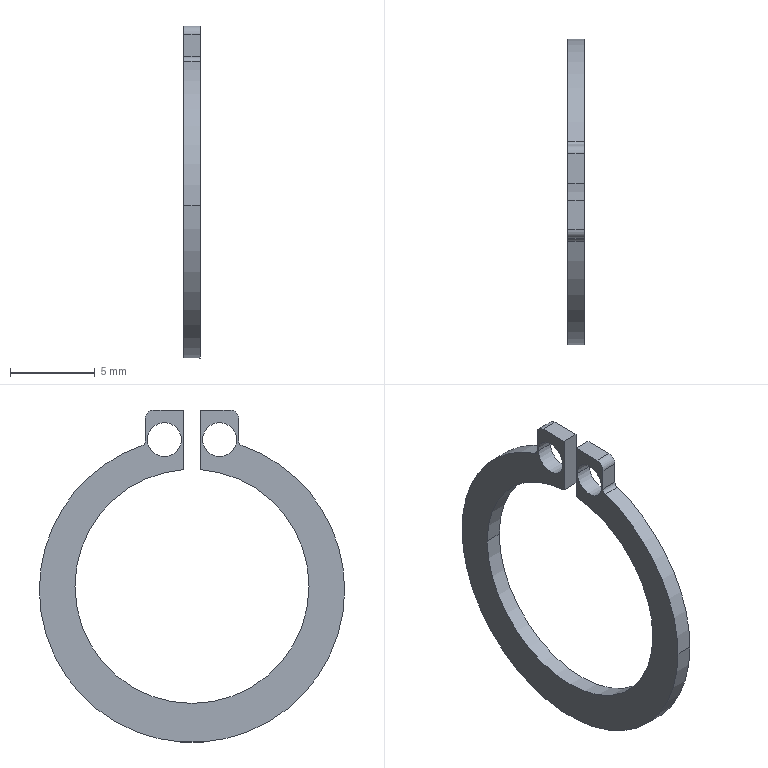Component | SolidWorks | CCD11-00TensioningAssembly-2_CCDAxisCard15-1 | 1 solid | 22 faces | box 1 x 18 x 19.6 mm | volume 105 mm3 | cylinder 14 | plane 8 | commonest cylinder face diameters 2 x4 18 x3 13.8 x3 1 x2 0.6 x2
build123d program:
from build123d import *

# Parameters (mm, degrees)
SKETCH1_R           = 1
BOSS_EXTRUDE1_DEPTH = 1


with BuildPart() as part:
    # Sketch1 → Boss-Extrude1 (new body)
    with BuildSketch(Plane.XY.offset(1)):
        with BuildLine():
            Line((2.75, -9.9), (2.75, -8.586))
            ThreePointArc((2.75, -8.586), (2.806, -8.412), (2.952, -8.302))
            ThreePointArc((2.952, -8.302), (0, 9.2), (-2.952, -8.302))
            ThreePointArc((-2.952, -8.302), (-2.806, -8.412), (-2.75, -8.586))
            Line((-2.75, -8.586), (-2.75, -9.9))
            ThreePointArc((-2.75, -9.9), (-2.604, -10.254), (-2.25, -10.4))
            Line((-2.25, -10.4), (-0.5, -10.4))
            Line((-0.5, -10.4), (-0.5, -6.882))
            ThreePointArc((-0.5, -6.882), (0, 6.9), (0.5, -6.882))
            Line((0.5, -6.882), (0.5, -10.4))
            Line((0.5, -10.4), (2.25, -10.4))
            ThreePointArc((2.25, -10.4), (2.604, -10.254), (2.75, -9.9))
        make_face()
        with Locations(Location((1.625, -8.65, 0), (0, 0, 180))):
            Circle(SKETCH1_R, mode=Mode.SUBTRACT)
        with Locations(Location((-1.625, -8.65, 0), (0, 0, 180))):
            Circle(SKETCH1_R, mode=Mode.SUBTRACT)
    extrude(amount=-BOSS_EXTRUDE1_DEPTH)


solid = part.part

# Placed as in the assembly
solid = solid.moved(Location((119.879, 107.251, 149), (-90, 90, 0)))
STEP:
#1=COLOUR_RGB('',0.7922,0.8196,0.9333);
#2=FILL_AREA_STYLE_COLOUR('',#1);
#3=FILL_AREA_STYLE('',(#2));
#4=SURFACE_STYLE_FILL_AREA(#3);
#5=SURFACE_SIDE_STYLE('',(#4));
#6=SURFACE_STYLE_USAGE(.BOTH.,#5);
#7=PRESENTATION_STYLE_ASSIGNMENT((#6));
#8=CARTESIAN_POINT('',(4.759,4.119,6.207));
#9=VERTEX_POINT('',#8);
#10=CARTESIAN_POINT('',(4.759,4.198,6.207));
#11=VERTEX_POINT('',#10);
#12=CARTESIAN_POINT('',(4.759,4.159,6.207));
#13=DIRECTION('',(-1.,-0.,0.));
#14=DIRECTION('',(0.,-1.,0.));
#15=AXIS2_PLACEMENT_3D('',#12,#13,#14);
#16=CIRCLE('',#15,0.03937);
#17=EDGE_CURVE('',#9,#11,#16,.T.);
#18=ORIENTED_EDGE('',*,*,#17,.F.);
#19=CARTESIAN_POINT('',(4.72,4.119,6.207));
#20=VERTEX_POINT('',#19);
#21=CARTESIAN_POINT('',(4.759,4.119,6.207));
#22=DIRECTION('',(-1.,-0.,0.));
#23=VECTOR('',#22,39.37);
#24=LINE('',#21,#23);
#25=EDGE_CURVE('',#9,#20,#24,.T.);
#26=ORIENTED_EDGE('',*,*,#25,.T.);
#27=CARTESIAN_POINT('',(4.72,4.198,6.207));
#28=VERTEX_POINT('',#27);
#29=CARTESIAN_POINT('',(4.72,4.159,6.207));
#30=DIRECTION('',(-1.,-0.,0.));
#31=DIRECTION('',(0.,-1.,0.));
#32=AXIS2_PLACEMENT_3D('',#29,#30,#31);
#33=CIRCLE('',#32,0.03937);
#34=EDGE_CURVE('',#20,#28,#33,.T.);
#35=ORIENTED_EDGE('',*,*,#34,.T.);
#36=CARTESIAN_POINT('',(4.759,4.198,6.207));
#37=DIRECTION('',(-1.,-0.,0.));
#38=VECTOR('',#37,39.37);
#39=LINE('',#36,#38);
#40=EDGE_CURVE('',#11,#28,#39,.T.);
#41=ORIENTED_EDGE('',*,*,#40,.F.);
#42=EDGE_LOOP('',(#18,#26,#35,#41));
#43=FACE_OUTER_BOUND('',#42,.T.);
#44=CARTESIAN_POINT('',(4.759,4.159,6.207));
#45=DIRECTION('',(-1.,-0.,0.));
#46=DIRECTION('',(0.,1.,0.));
#47=AXIS2_PLACEMENT_3D('',#44,#45,#46);
#48=CYLINDRICAL_SURFACE('',#47,0.03937);
#49=ADVANCED_FACE('',(#43),#48,.F.);
#50=CARTESIAN_POINT('',(4.759,4.247,6.207));
#51=VERTEX_POINT('',#50);
#52=CARTESIAN_POINT('',(4.759,4.326,6.207));
#53=VERTEX_POINT('',#52);
#54=CARTESIAN_POINT('',(4.759,4.286,6.207));
#55=DIRECTION('',(-1.,-0.,0.));
#56=DIRECTION('',(0.,-1.,0.));
#57=AXIS2_PLACEMENT_3D('',#54,#55,#56);
#58=CIRCLE('',#57,0.03937);
#59=EDGE_CURVE('',#51,#53,#58,.T.);
#60=ORIENTED_EDGE('',*,*,#59,.F.);
#61=CARTESIAN_POINT('',(4.72,4.247,6.207));
#62=VERTEX_POINT('',#61);
#63=CARTESIAN_POINT('',(4.759,4.247,6.207));
#64=DIRECTION('',(-1.,-0.,0.));
#65=VECTOR('',#64,39.37);
#66=LINE('',#63,#65);
#67=EDGE_CURVE('',#51,#62,#66,.T.);
#68=ORIENTED_EDGE('',*,*,#67,.T.);
#69=CARTESIAN_POINT('',(4.72,4.326,6.207));
#70=VERTEX_POINT('',#69);
#71=CARTESIAN_POINT('',(4.72,4.286,6.207));
#72=DIRECTION('',(-1.,-0.,0.));
#73=DIRECTION('',(0.,-1.,0.));
#74=AXIS2_PLACEMENT_3D('',#71,#72,#73);
#75=CIRCLE('',#74,0.03937);
#76=EDGE_CURVE('',#62,#70,#75,.T.);
#77=ORIENTED_EDGE('',*,*,#76,.T.);
#78=CARTESIAN_POINT('',(4.759,4.326,6.207));
#79=DIRECTION('',(-1.,-0.,0.));
#80=VECTOR('',#79,39.37);
#81=LINE('',#78,#80);
#82=EDGE_CURVE('',#53,#70,#81,.T.);
#83=ORIENTED_EDGE('',*,*,#82,.F.);
#84=EDGE_LOOP('',(#60,#68,#77,#83));
#85=FACE_OUTER_BOUND('',#84,.T.);
#86=CARTESIAN_POINT('',(4.759,4.286,6.207));
#87=DIRECTION('',(-1.,-0.,0.));
#88=DIRECTION('',(0.,1.,0.));
#89=AXIS2_PLACEMENT_3D('',#86,#87,#88);
#90=CYLINDRICAL_SURFACE('',#89,0.03937);
#91=ADVANCED_FACE('',(#85),#90,.F.);
#92=CARTESIAN_POINT('',(4.759,4.577,5.858));
#93=VERTEX_POINT('',#92);
#94=CARTESIAN_POINT('',(4.759,3.868,5.858));
#95=VERTEX_POINT('',#94);
#96=CARTESIAN_POINT('',(4.759,4.222,5.858));
#97=DIRECTION('',(-1.,-0.,0.));
#98=DIRECTION('',(-0.,1.,0.));
#99=AXIS2_PLACEMENT_3D('',#96,#97,#98);
#100=CIRCLE('',#99,0.3543);
#101=EDGE_CURVE('',#93,#95,#100,.T.);
#102=ORIENTED_EDGE('',*,*,#101,.T.);
#103=CARTESIAN_POINT('',(4.72,3.868,5.858));
#104=VERTEX_POINT('',#103);
#105=CARTESIAN_POINT('',(4.759,3.868,5.858));
#106=DIRECTION('',(-1.,-0.,0.));
#107=VECTOR('',#106,39.37);
#108=LINE('',#105,#107);
#109=EDGE_CURVE('',#95,#104,#108,.T.);
#110=ORIENTED_EDGE('',*,*,#109,.T.);
#111=CARTESIAN_POINT('',(4.72,4.577,5.858));
#112=VERTEX_POINT('',#111);
#113=CARTESIAN_POINT('',(4.72,4.222,5.858));
#114=DIRECTION('',(-1.,-0.,0.));
#115=DIRECTION('',(-0.,1.,0.));
#116=AXIS2_PLACEMENT_3D('',#113,#114,#115);
#117=CIRCLE('',#116,0.3543);
#118=EDGE_CURVE('',#112,#104,#117,.T.);
#119=ORIENTED_EDGE('',*,*,#118,.F.);
#120=CARTESIAN_POINT('',(4.759,4.577,5.858));
#121=DIRECTION('',(-1.,-0.,0.));
#122=VECTOR('',#121,39.37);
#123=LINE('',#120,#122);
#124=EDGE_CURVE('',#93,#112,#123,.T.);
#125=ORIENTED_EDGE('',*,*,#124,.F.);
#126=EDGE_LOOP('',(#102,#110,#119,#125));
#127=FACE_OUTER_BOUND('',#126,.T.);
#128=CARTESIAN_POINT('',(4.759,4.222,5.858));
#129=DIRECTION('',(-1.,-0.,0.));
#130=DIRECTION('',(-0.,1.,0.));
#131=AXIS2_PLACEMENT_3D('',#128,#129,#130);
#132=CYLINDRICAL_SURFACE('',#131,0.3543);
#133=ADVANCED_FACE('',(#127),#132,.T.);
#134=CARTESIAN_POINT('',(4.759,4.339,6.193));
#135=VERTEX_POINT('',#134);
#136=CARTESIAN_POINT('',(4.759,4.222,5.858));
#137=DIRECTION('',(-1.,-0.,0.));
#138=DIRECTION('',(-0.,1.,0.));
#139=AXIS2_PLACEMENT_3D('',#136,#137,#138);
#140=CIRCLE('',#139,0.3543);
#141=EDGE_CURVE('',#135,#93,#140,.T.);
#142=ORIENTED_EDGE('',*,*,#141,.T.);
#143=ORIENTED_EDGE('',*,*,#124,.T.);
#144=CARTESIAN_POINT('',(4.72,4.339,6.193));
#145=VERTEX_POINT('',#144);
#146=CARTESIAN_POINT('',(4.72,4.222,5.858));
#147=DIRECTION('',(-1.,-0.,0.));
#148=DIRECTION('',(-0.,1.,0.));
#149=AXIS2_PLACEMENT_3D('',#146,#147,#148);
#150=CIRCLE('',#149,0.3543);
#151=EDGE_CURVE('',#145,#112,#150,.T.);
#152=ORIENTED_EDGE('',*,*,#151,.F.);
#153=CARTESIAN_POINT('',(4.759,4.339,6.193));
#154=DIRECTION('',(-1.,-0.,0.));
#155=VECTOR('',#154,39.37);
#156=LINE('',#153,#155);
#157=EDGE_CURVE('',#135,#145,#156,.T.);
#158=ORIENTED_EDGE('',*,*,#157,.F.);
#159=EDGE_LOOP('',(#142,#143,#152,#158));
#160=FACE_OUTER_BOUND('',#159,.T.);
#161=CARTESIAN_POINT('',(4.759,4.222,5.858));
#162=DIRECTION('',(-1.,-0.,0.));
#163=DIRECTION('',(-0.,1.,0.));
#164=AXIS2_PLACEMENT_3D('',#161,#162,#163);
#165=CYLINDRICAL_SURFACE('',#164,0.3543);
#166=ADVANCED_FACE('',(#160),#165,.T.);
#167=CARTESIAN_POINT('',(4.759,4.203,6.137));
#168=VERTEX_POINT('',#167);
#169=CARTESIAN_POINT('',(4.759,3.951,5.866));
#170=VERTEX_POINT('',#169);
#171=CARTESIAN_POINT('',(4.759,4.222,5.866));
#172=DIRECTION('',(1.,0.,-0.));
#173=DIRECTION('',(0.,-1.,0.));
#174=AXIS2_PLACEMENT_3D('',#171,#172,#173);
#175=CIRCLE('',#174,0.2717);
#176=EDGE_CURVE('',#168,#170,#175,.T.);
#177=ORIENTED_EDGE('',*,*,#176,.T.);
#178=CARTESIAN_POINT('',(4.72,3.951,5.866));
#179=VERTEX_POINT('',#178);
#180=CARTESIAN_POINT('',(4.759,3.951,5.866));
#181=DIRECTION('',(-1.,-0.,0.));
#182=VECTOR('',#181,39.37);
#183=LINE('',#180,#182);
#184=EDGE_CURVE('',#170,#179,#183,.T.);
#185=ORIENTED_EDGE('',*,*,#184,.T.);
#186=CARTESIAN_POINT('',(4.72,4.203,6.137));
#187=VERTEX_POINT('',#186);
#188=CARTESIAN_POINT('',(4.72,4.222,5.866));
#189=DIRECTION('',(1.,0.,-0.));
#190=DIRECTION('',(0.,-1.,0.));
#191=AXIS2_PLACEMENT_3D('',#188,#189,#190);
#192=CIRCLE('',#191,0.2717);
#193=EDGE_CURVE('',#187,#179,#192,.T.);
#194=ORIENTED_EDGE('',*,*,#193,.F.);
#195=CARTESIAN_POINT('',(4.759,4.203,6.137));
#196=DIRECTION('',(-1.,-0.,0.));
#197=VECTOR('',#196,39.37);
#198=LINE('',#195,#197);
#199=EDGE_CURVE('',#168,#187,#198,.T.);
#200=ORIENTED_EDGE('',*,*,#199,.F.);
#201=EDGE_LOOP('',(#177,#185,#194,#200));
#202=FACE_OUTER_BOUND('',#201,.T.);
#203=CARTESIAN_POINT('',(4.759,4.222,5.866));
#204=DIRECTION('',(-1.,-0.,0.));
#205=DIRECTION('',(-0.,1.,0.));
#206=AXIS2_PLACEMENT_3D('',#203,#204,#205);
#207=CYLINDRICAL_SURFACE('',#206,0.2717);
#208=ADVANCED_FACE('',(#202),#207,.F.);
#209=ORIENTED_EDGE('',*,*,#184,.F.);
#210=CARTESIAN_POINT('',(4.759,4.494,5.866));
#211=VERTEX_POINT('',#210);
#212=CARTESIAN_POINT('',(4.759,4.222,5.866));
#213=DIRECTION('',(1.,0.,-0.));
#214=DIRECTION('',(0.,-1.,0.));
#215=AXIS2_PLACEMENT_3D('',#212,#213,#214);
#216=CIRCLE('',#215,0.2717);
#217=EDGE_CURVE('',#170,#211,#216,.T.);
#218=ORIENTED_EDGE('',*,*,#217,.T.);
#219=CARTESIAN_POINT('',(4.72,4.494,5.866));
#220=VERTEX_POINT('',#219);
#221=CARTESIAN_POINT('',(4.759,4.494,5.866));
#222=DIRECTION('',(-1.,-0.,0.));
#223=VECTOR('',#222,39.37);
#224=LINE('',#221,#223);
#225=EDGE_CURVE('',#211,#220,#224,.T.);
#226=ORIENTED_EDGE('',*,*,#225,.T.);
#227=CARTESIAN_POINT('',(4.72,4.222,5.866));
#228=DIRECTION('',(1.,0.,-0.));
#229=DIRECTION('',(0.,-1.,0.));
#230=AXIS2_PLACEMENT_3D('',#227,#228,#229);
#231=CIRCLE('',#230,0.2717);
#232=EDGE_CURVE('',#179,#220,#231,.T.);
#233=ORIENTED_EDGE('',*,*,#232,.F.);
#234=EDGE_LOOP('',(#209,#218,#226,#233));
#235=FACE_OUTER_BOUND('',#234,.T.);
#236=CARTESIAN_POINT('',(4.759,4.222,5.866));
#237=DIRECTION('',(-1.,-0.,0.));
#238=DIRECTION('',(-0.,1.,0.));
#239=AXIS2_PLACEMENT_3D('',#236,#237,#238);
#240=CYLINDRICAL_SURFACE('',#239,0.2717);
#241=ADVANCED_FACE('',(#235),#240,.F.);
#242=CARTESIAN_POINT('',(4.72,4.311,6.276));
#243=VERTEX_POINT('',#242);
#244=CARTESIAN_POINT('',(4.72,4.331,6.256));
#245=VERTEX_POINT('',#244);
#246=CARTESIAN_POINT('',(4.72,4.311,6.256));
#247=DIRECTION('',(-1.,-0.,0.));
#248=DIRECTION('',(0.,1.,0.));
#249=AXIS2_PLACEMENT_3D('',#246,#247,#248);
#250=CIRCLE('',#249,0.01969);
#251=EDGE_CURVE('',#243,#245,#250,.T.);
#252=ORIENTED_EDGE('',*,*,#251,.F.);
#253=CARTESIAN_POINT('',(4.759,4.311,6.276));
#254=VERTEX_POINT('',#253);
#255=CARTESIAN_POINT('',(4.759,4.311,6.276));
#256=DIRECTION('',(-1.,-0.,0.));
#257=VECTOR('',#256,39.37);
#258=LINE('',#255,#257);
#259=EDGE_CURVE('',#254,#243,#258,.T.);
#260=ORIENTED_EDGE('',*,*,#259,.F.);
#261=CARTESIAN_POINT('',(4.759,4.331,6.256));
#262=VERTEX_POINT('',#261);
#263=CARTESIAN_POINT('',(4.759,4.311,6.256));
#264=DIRECTION('',(-1.,-0.,0.));
#265=DIRECTION('',(0.,1.,0.));
#266=AXIS2_PLACEMENT_3D('',#263,#264,#265);
#267=CIRCLE('',#266,0.01969);
#268=EDGE_CURVE('',#254,#262,#267,.T.);
#269=ORIENTED_EDGE('',*,*,#268,.T.);
#270=CARTESIAN_POINT('',(4.759,4.331,6.256));
#271=DIRECTION('',(-1.,-0.,0.));
#272=VECTOR('',#271,39.37);
#273=LINE('',#270,#272);
#274=EDGE_CURVE('',#262,#245,#273,.T.);
#275=ORIENTED_EDGE('',*,*,#274,.T.);
#276=EDGE_LOOP('',(#252,#260,#269,#275));
#277=FACE_OUTER_BOUND('',#276,.T.);
#278=CARTESIAN_POINT('',(4.759,4.311,6.256));
#279=DIRECTION('',(-1.,-0.,0.));
#280=DIRECTION('',(0.,1.,0.));
#281=AXIS2_PLACEMENT_3D('',#278,#279,#280);
#282=CYLINDRICAL_SURFACE('',#281,0.01969);
#283=ADVANCED_FACE('',(#277),#282,.T.);
#284=CARTESIAN_POINT('',(4.72,4.242,6.276));
#285=VERTEX_POINT('',#284);
#286=CARTESIAN_POINT('',(4.72,4.242,6.276));
#287=DIRECTION('',(-0.,1.,0.));
#288=VECTOR('',#287,39.37);
#289=LINE('',#286,#288);
#290=EDGE_CURVE('',#285,#243,#289,.T.);
#291=ORIENTED_EDGE('',*,*,#290,.F.);
#292=CARTESIAN_POINT('',(4.759,4.242,6.276));
#293=VERTEX_POINT('',#292);
#294=CARTESIAN_POINT('',(4.759,4.242,6.276));
#295=DIRECTION('',(-1.,-0.,0.));
#296=VECTOR('',#295,39.37);
#297=LINE('',#294,#296);
#298=EDGE_CURVE('',#293,#285,#297,.T.);
#299=ORIENTED_EDGE('',*,*,#298,.F.);
#300=CARTESIAN_POINT('',(4.759,4.242,6.276));
#301=DIRECTION('',(-0.,1.,0.));
#302=VECTOR('',#301,39.37);
#303=LINE('',#300,#302);
#304=EDGE_CURVE('',#293,#254,#303,.T.);
#305=ORIENTED_EDGE('',*,*,#304,.T.);
#306=ORIENTED_EDGE('',*,*,#259,.T.);
#307=EDGE_LOOP('',(#291,#299,#305,#306));
#308=FACE_OUTER_BOUND('',#307,.T.);
#309=CARTESIAN_POINT('',(4.759,4.242,6.276));
#310=DIRECTION('',(0.,-0.,1.));
#311=DIRECTION('',(-0.,1.,0.));
#312=AXIS2_PLACEMENT_3D('',#309,#310,#311);
#313=PLANE('',#312);
#314=ADVANCED_FACE('',(#308),#313,.T.);
#315=CARTESIAN_POINT('',(4.72,4.242,6.137));
#316=VERTEX_POINT('',#315);
#317=CARTESIAN_POINT('',(4.72,4.242,6.137));
#318=DIRECTION('',(0.,-0.,1.));
#319=VECTOR('',#318,39.37);
#320=LINE('',#317,#319);
#321=EDGE_CURVE('',#316,#285,#320,.T.);
#322=ORIENTED_EDGE('',*,*,#321,.F.);
#323=CARTESIAN_POINT('',(4.759,4.242,6.137));
#324=VERTEX_POINT('',#323);
#325=CARTESIAN_POINT('',(4.759,4.242,6.137));
#326=DIRECTION('',(-1.,-0.,0.));
#327=VECTOR('',#326,39.37);
#328=LINE('',#325,#327);
#329=EDGE_CURVE('',#324,#316,#328,.T.);
#330=ORIENTED_EDGE('',*,*,#329,.F.);
#331=CARTESIAN_POINT('',(4.759,4.242,6.137));
#332=DIRECTION('',(0.,-0.,1.));
#333=VECTOR('',#332,39.37);
#334=LINE('',#331,#333);
#335=EDGE_CURVE('',#324,#293,#334,.T.);
#336=ORIENTED_EDGE('',*,*,#335,.T.);
#337=ORIENTED_EDGE('',*,*,#298,.T.);
#338=EDGE_LOOP('',(#322,#330,#336,#337));
#339=FACE_OUTER_BOUND('',#338,.T.);
#340=CARTESIAN_POINT('',(4.759,4.242,6.137));
#341=DIRECTION('',(0.,-1.,-0.));
#342=DIRECTION('',(0.,-0.,1.));
#343=AXIS2_PLACEMENT_3D('',#340,#341,#342);
#344=PLANE('',#343);
#345=ADVANCED_FACE('',(#339),#344,.T.);
#346=ORIENTED_EDGE('',*,*,#225,.F.);
#347=CARTESIAN_POINT('',(4.759,4.222,5.866));
#348=DIRECTION('',(1.,0.,-0.));
#349=DIRECTION('',(0.,-1.,0.));
#350=AXIS2_PLACEMENT_3D('',#347,#348,#349);
#351=CIRCLE('',#350,0.2717);
#352=EDGE_CURVE('',#211,#324,#351,.T.);
#353=ORIENTED_EDGE('',*,*,#352,.T.);
#354=ORIENTED_EDGE('',*,*,#329,.T.);
#355=CARTESIAN_POINT('',(4.72,4.222,5.866));
#356=DIRECTION('',(1.,0.,-0.));
#357=DIRECTION('',(0.,-1.,0.));
#358=AXIS2_PLACEMENT_3D('',#355,#356,#357);
#359=CIRCLE('',#358,0.2717);
#360=EDGE_CURVE('',#220,#316,#359,.T.);
#361=ORIENTED_EDGE('',*,*,#360,.F.);
#362=EDGE_LOOP('',(#346,#353,#354,#361));
#363=FACE_OUTER_BOUND('',#362,.T.);
#364=CARTESIAN_POINT('',(4.759,4.222,5.866));
#365=DIRECTION('',(-1.,-0.,0.));
#366=DIRECTION('',(-0.,1.,0.));
#367=AXIS2_PLACEMENT_3D('',#364,#365,#366);
#368=CYLINDRICAL_SURFACE('',#367,0.2717);
#369=ADVANCED_FACE('',(#363),#368,.F.);
#370=CARTESIAN_POINT('',(4.72,4.203,6.276));
#371=VERTEX_POINT('',#370);
#372=CARTESIAN_POINT('',(4.72,4.203,6.276));
#373=DIRECTION('',(-0.,-0.,-1.));
#374=VECTOR('',#373,39.37);
#375=LINE('',#372,#374);
#376=EDGE_CURVE('',#371,#187,#375,.T.);
#377=ORIENTED_EDGE('',*,*,#376,.F.);
#378=CARTESIAN_POINT('',(4.759,4.203,6.276));
#379=VERTEX_POINT('',#378);
#380=CARTESIAN_POINT('',(4.759,4.203,6.276));
#381=DIRECTION('',(-1.,-0.,0.));
#382=VECTOR('',#381,39.37);
#383=LINE('',#380,#382);
#384=EDGE_CURVE('',#379,#371,#383,.T.);
#385=ORIENTED_EDGE('',*,*,#384,.F.);
#386=CARTESIAN_POINT('',(4.759,4.203,6.276));
#387=DIRECTION('',(-0.,-0.,-1.));
#388=VECTOR('',#387,39.37);
#389=LINE('',#386,#388);
#390=EDGE_CURVE('',#379,#168,#389,.T.);
#391=ORIENTED_EDGE('',*,*,#390,.T.);
#392=ORIENTED_EDGE('',*,*,#199,.T.);
#393=EDGE_LOOP('',(#377,#385,#391,#392));
#394=FACE_OUTER_BOUND('',#393,.T.);
#395=CARTESIAN_POINT('',(4.759,4.203,6.276));
#396=DIRECTION('',(-0.,1.,-0.));
#397=DIRECTION('',(-0.,-0.,-1.));
#398=AXIS2_PLACEMENT_3D('',#395,#396,#397);
#399=PLANE('',#398);
#400=ADVANCED_FACE('',(#394),#399,.T.);
#401=CARTESIAN_POINT('',(4.72,4.134,6.276));
#402=VERTEX_POINT('',#401);
#403=CARTESIAN_POINT('',(4.72,4.134,6.276));
#404=DIRECTION('',(-0.,1.,0.));
#405=VECTOR('',#404,39.37);
#406=LINE('',#403,#405);
#407=EDGE_CURVE('',#402,#371,#406,.T.);
#408=ORIENTED_EDGE('',*,*,#407,.F.);
#409=CARTESIAN_POINT('',(4.759,4.134,6.276));
#410=VERTEX_POINT('',#409);
#411=CARTESIAN_POINT('',(4.759,4.134,6.276));
#412=DIRECTION('',(-1.,-0.,0.));
#413=VECTOR('',#412,39.37);
#414=LINE('',#411,#413);
#415=EDGE_CURVE('',#410,#402,#414,.T.);
#416=ORIENTED_EDGE('',*,*,#415,.F.);
#417=CARTESIAN_POINT('',(4.759,4.134,6.276));
#418=DIRECTION('',(-0.,1.,0.));
#419=VECTOR('',#418,39.37);
#420=LINE('',#417,#419);
#421=EDGE_CURVE('',#410,#379,#420,.T.);
#422=ORIENTED_EDGE('',*,*,#421,.T.);
#423=ORIENTED_EDGE('',*,*,#384,.T.);
#424=EDGE_LOOP('',(#408,#416,#422,#423));
#425=FACE_OUTER_BOUND('',#424,.T.);
#426=CARTESIAN_POINT('',(4.759,4.134,6.276));
#427=DIRECTION('',(0.,-0.,1.));
#428=DIRECTION('',(1.,0.,-0.));
#429=AXIS2_PLACEMENT_3D('',#426,#427,#428);
#430=PLANE('',#429);
#431=ADVANCED_FACE('',(#425),#430,.T.);
#432=CARTESIAN_POINT('',(4.72,4.114,6.256));
#433=VERTEX_POINT('',#432);
#434=CARTESIAN_POINT('',(4.72,4.134,6.256));
#435=DIRECTION('',(-1.,-0.,0.));
#436=DIRECTION('',(0.,1.,0.));
#437=AXIS2_PLACEMENT_3D('',#434,#435,#436);
#438=CIRCLE('',#437,0.01969);
#439=EDGE_CURVE('',#433,#402,#438,.T.);
#440=ORIENTED_EDGE('',*,*,#439,.F.);
#441=CARTESIAN_POINT('',(4.759,4.114,6.256));
#442=VERTEX_POINT('',#441);
#443=CARTESIAN_POINT('',(4.759,4.114,6.256));
#444=DIRECTION('',(-1.,-0.,0.));
#445=VECTOR('',#444,39.37);
#446=LINE('',#443,#445);
#447=EDGE_CURVE('',#442,#433,#446,.T.);
#448=ORIENTED_EDGE('',*,*,#447,.F.);
#449=CARTESIAN_POINT('',(4.759,4.134,6.256));
#450=DIRECTION('',(-1.,-0.,0.));
#451=DIRECTION('',(0.,1.,0.));
#452=AXIS2_PLACEMENT_3D('',#449,#450,#451);
#453=CIRCLE('',#452,0.01969);
#454=EDGE_CURVE('',#442,#410,#453,.T.);
#455=ORIENTED_EDGE('',*,*,#454,.T.);
#456=ORIENTED_EDGE('',*,*,#415,.T.);
#457=EDGE_LOOP('',(#440,#448,#455,#456));
#458=FACE_OUTER_BOUND('',#457,.T.);
#459=CARTESIAN_POINT('',(4.759,4.134,6.256));
#460=DIRECTION('',(-1.,-0.,0.));
#461=DIRECTION('',(0.,1.,0.));
#462=AXIS2_PLACEMENT_3D('',#459,#460,#461);
#463=CYLINDRICAL_SURFACE('',#462,0.01969);
#464=ADVANCED_FACE('',(#458),#463,.T.);
#465=CARTESIAN_POINT('',(4.72,4.114,6.204));
#466=VERTEX_POINT('',#465);
#467=CARTESIAN_POINT('',(4.72,4.114,6.204));
#468=DIRECTION('',(0.,-0.,1.));
#469=VECTOR('',#468,39.37);
#470=LINE('',#467,#469);
#471=EDGE_CURVE('',#466,#433,#470,.T.);
#472=ORIENTED_EDGE('',*,*,#471,.F.);
#473=CARTESIAN_POINT('',(4.759,4.114,6.204));
#474=VERTEX_POINT('',#473);
#475=CARTESIAN_POINT('',(4.759,4.114,6.204));
#476=DIRECTION('',(-1.,-0.,0.));
#477=VECTOR('',#476,39.37);
#478=LINE('',#475,#477);
#479=EDGE_CURVE('',#474,#466,#478,.T.);
#480=ORIENTED_EDGE('',*,*,#479,.F.);
#481=CARTESIAN_POINT('',(4.759,4.114,6.204));
#482=DIRECTION('',(0.,-0.,1.));
#483=VECTOR('',#482,39.37);
#484=LINE('',#481,#483);
#485=EDGE_CURVE('',#474,#442,#484,.T.);
#486=ORIENTED_EDGE('',*,*,#485,.T.);
#487=ORIENTED_EDGE('',*,*,#447,.T.);
#488=EDGE_LOOP('',(#472,#480,#486,#487));
#489=FACE_OUTER_BOUND('',#488,.T.);
#490=CARTESIAN_POINT('',(4.759,4.114,6.204));
#491=DIRECTION('',(0.,-1.,-0.));
#492=DIRECTION('',(0.,-0.,1.));
#493=AXIS2_PLACEMENT_3D('',#490,#491,#492);
#494=PLANE('',#493);
#495=ADVANCED_FACE('',(#489),#494,.T.);
#496=CARTESIAN_POINT('',(4.72,4.106,6.193));
#497=VERTEX_POINT('',#496);
#498=CARTESIAN_POINT('',(4.72,4.102,6.204));
#499=DIRECTION('',(1.,0.,-0.));
#500=DIRECTION('',(0.,-1.,0.));
#501=AXIS2_PLACEMENT_3D('',#498,#499,#500);
#502=CIRCLE('',#501,0.01181);
#503=EDGE_CURVE('',#497,#466,#502,.T.);
#504=ORIENTED_EDGE('',*,*,#503,.F.);
#505=CARTESIAN_POINT('',(4.759,4.106,6.193));
#506=VERTEX_POINT('',#505);
#507=CARTESIAN_POINT('',(4.759,4.106,6.193));
#508=DIRECTION('',(-1.,-0.,0.));
#509=VECTOR('',#508,39.37);
#510=LINE('',#507,#509);
#511=EDGE_CURVE('',#506,#497,#510,.T.);
#512=ORIENTED_EDGE('',*,*,#511,.F.);
#513=CARTESIAN_POINT('',(4.759,4.102,6.204));
#514=DIRECTION('',(1.,0.,-0.));
#515=DIRECTION('',(0.,-1.,0.));
#516=AXIS2_PLACEMENT_3D('',#513,#514,#515);
#517=CIRCLE('',#516,0.01181);
#518=EDGE_CURVE('',#506,#474,#517,.T.);
#519=ORIENTED_EDGE('',*,*,#518,.T.);
#520=ORIENTED_EDGE('',*,*,#479,.T.);
#521=EDGE_LOOP('',(#504,#512,#519,#520));
#522=FACE_OUTER_BOUND('',#521,.T.);
#523=CARTESIAN_POINT('',(4.759,4.102,6.204));
#524=DIRECTION('',(-1.,-0.,0.));
#525=DIRECTION('',(0.,1.,0.));
#526=AXIS2_PLACEMENT_3D('',#523,#524,#525);
#527=CYLINDRICAL_SURFACE('',#526,0.01181);
#528=ADVANCED_FACE('',(#522),#527,.F.);
#529=ORIENTED_EDGE('',*,*,#109,.F.);
#530=CARTESIAN_POINT('',(4.759,4.222,5.858));
#531=DIRECTION('',(-1.,-0.,0.));
#532=DIRECTION('',(-0.,1.,0.));
#533=AXIS2_PLACEMENT_3D('',#530,#531,#532);
#534=CIRCLE('',#533,0.3543);
#535=EDGE_CURVE('',#95,#506,#534,.T.);
#536=ORIENTED_EDGE('',*,*,#535,.T.);
#537=ORIENTED_EDGE('',*,*,#511,.T.);
#538=CARTESIAN_POINT('',(4.72,4.222,5.858));
#539=DIRECTION('',(-1.,-0.,0.));
#540=DIRECTION('',(-0.,1.,0.));
#541=AXIS2_PLACEMENT_3D('',#538,#539,#540);
#542=CIRCLE('',#541,0.3543);
#543=EDGE_CURVE('',#104,#497,#542,.T.);
#544=ORIENTED_EDGE('',*,*,#543,.F.);
#545=EDGE_LOOP('',(#529,#536,#537,#544));
#546=FACE_OUTER_BOUND('',#545,.T.);
#547=CARTESIAN_POINT('',(4.759,4.222,5.858));
#548=DIRECTION('',(-1.,-0.,0.));
#549=DIRECTION('',(-0.,1.,0.));
#550=AXIS2_PLACEMENT_3D('',#547,#548,#549);
#551=CYLINDRICAL_SURFACE('',#550,0.3543);
#552=ADVANCED_FACE('',(#546),#551,.T.);
#553=CARTESIAN_POINT('',(4.72,4.331,6.204));
#554=VERTEX_POINT('',#553);
#555=CARTESIAN_POINT('',(4.72,4.343,6.204));
#556=DIRECTION('',(1.,0.,-0.));
#557=DIRECTION('',(0.,-1.,0.));
#558=AXIS2_PLACEMENT_3D('',#555,#556,#557);
#559=CIRCLE('',#558,0.01181);
#560=EDGE_CURVE('',#554,#145,#559,.T.);
#561=ORIENTED_EDGE('',*,*,#560,.F.);
#562=CARTESIAN_POINT('',(4.759,4.331,6.204));
#563=VERTEX_POINT('',#562);
#564=CARTESIAN_POINT('',(4.759,4.331,6.204));
#565=DIRECTION('',(-1.,-0.,0.));
#566=VECTOR('',#565,39.37);
#567=LINE('',#564,#566);
#568=EDGE_CURVE('',#563,#554,#567,.T.);
#569=ORIENTED_EDGE('',*,*,#568,.F.);
#570=CARTESIAN_POINT('',(4.759,4.343,6.204));
#571=DIRECTION('',(1.,0.,-0.));
#572=DIRECTION('',(0.,-1.,0.));
#573=AXIS2_PLACEMENT_3D('',#570,#571,#572);
#574=CIRCLE('',#573,0.01181);
#575=EDGE_CURVE('',#563,#135,#574,.T.);
#576=ORIENTED_EDGE('',*,*,#575,.T.);
#577=ORIENTED_EDGE('',*,*,#157,.T.);
#578=EDGE_LOOP('',(#561,#569,#576,#577));
#579=FACE_OUTER_BOUND('',#578,.T.);
#580=CARTESIAN_POINT('',(4.759,4.343,6.204));
#581=DIRECTION('',(-1.,-0.,0.));
#582=DIRECTION('',(0.,1.,0.));
#583=AXIS2_PLACEMENT_3D('',#580,#581,#582);
#584=CYLINDRICAL_SURFACE('',#583,0.01181);
#585=ADVANCED_FACE('',(#579),#584,.F.);
#586=CARTESIAN_POINT('',(4.72,4.331,6.256));
#587=DIRECTION('',(-0.,-0.,-1.));
#588=VECTOR('',#587,39.37);
#589=LINE('',#586,#588);
#590=EDGE_CURVE('',#245,#554,#589,.T.);
#591=ORIENTED_EDGE('',*,*,#590,.F.);
#592=ORIENTED_EDGE('',*,*,#274,.F.);
#593=CARTESIAN_POINT('',(4.759,4.331,6.256));
#594=DIRECTION('',(-0.,-0.,-1.));
#595=VECTOR('',#594,39.37);
#596=LINE('',#593,#595);
#597=EDGE_CURVE('',#262,#563,#596,.T.);
#598=ORIENTED_EDGE('',*,*,#597,.T.);
#599=ORIENTED_EDGE('',*,*,#568,.T.);
#600=EDGE_LOOP('',(#591,#592,#598,#599));
#601=FACE_OUTER_BOUND('',#600,.T.);
#602=CARTESIAN_POINT('',(4.759,4.331,6.256));
#603=DIRECTION('',(-0.,1.,-0.));
#604=DIRECTION('',(-0.,-0.,-1.));
#605=AXIS2_PLACEMENT_3D('',#602,#603,#604);
#606=PLANE('',#605);
#607=ADVANCED_FACE('',(#601),#606,.T.);
#608=CARTESIAN_POINT('',(4.759,4.159,6.207));
#609=DIRECTION('',(-1.,-0.,0.));
#610=DIRECTION('',(0.,-1.,0.));
#611=AXIS2_PLACEMENT_3D('',#608,#609,#610);
#612=CIRCLE('',#611,0.03937);
#613=EDGE_CURVE('',#11,#9,#612,.T.);
#614=ORIENTED_EDGE('',*,*,#613,.T.);
#615=ORIENTED_EDGE('',*,*,#17,.T.);
#616=EDGE_LOOP('',(#614,#615));
#617=FACE_BOUND('',#616,.T.);
#618=CARTESIAN_POINT('',(4.759,4.286,6.207));
#619=DIRECTION('',(-1.,-0.,0.));
#620=DIRECTION('',(0.,-1.,0.));
#621=AXIS2_PLACEMENT_3D('',#618,#619,#620);
#622=CIRCLE('',#621,0.03937);
#623=EDGE_CURVE('',#53,#51,#622,.T.);
#624=ORIENTED_EDGE('',*,*,#623,.T.);
#625=ORIENTED_EDGE('',*,*,#59,.T.);
#626=EDGE_LOOP('',(#624,#625));
#627=FACE_BOUND('',#626,.T.);
#628=ORIENTED_EDGE('',*,*,#268,.F.);
#629=ORIENTED_EDGE('',*,*,#304,.F.);
#630=ORIENTED_EDGE('',*,*,#335,.F.);
#631=ORIENTED_EDGE('',*,*,#352,.F.);
#632=ORIENTED_EDGE('',*,*,#217,.F.);
#633=ORIENTED_EDGE('',*,*,#176,.F.);
#634=ORIENTED_EDGE('',*,*,#390,.F.);
#635=ORIENTED_EDGE('',*,*,#421,.F.);
#636=ORIENTED_EDGE('',*,*,#454,.F.);
#637=ORIENTED_EDGE('',*,*,#485,.F.);
#638=ORIENTED_EDGE('',*,*,#518,.F.);
#639=ORIENTED_EDGE('',*,*,#535,.F.);
#640=ORIENTED_EDGE('',*,*,#101,.F.);
#641=ORIENTED_EDGE('',*,*,#141,.F.);
#642=ORIENTED_EDGE('',*,*,#575,.F.);
#643=ORIENTED_EDGE('',*,*,#597,.F.);
#644=EDGE_LOOP('',(#628,#629,#630,#631,#632,#633,#634,#635,#636,#637,#638,#639,#640,#641,#642,#643));
#645=FACE_OUTER_BOUND('',#644,.T.);
#646=CARTESIAN_POINT('',(4.759,4.311,6.256));
#647=DIRECTION('',(-1.,-0.,0.));
#648=DIRECTION('',(-0.,1.,0.));
#649=AXIS2_PLACEMENT_3D('',#646,#647,#648);
#650=PLANE('',#649);
#651=ADVANCED_FACE('',(#617,#627,#645),#650,.F.);
#652=CARTESIAN_POINT('',(4.72,4.159,6.207));
#653=DIRECTION('',(-1.,-0.,0.));
#654=DIRECTION('',(0.,-1.,0.));
#655=AXIS2_PLACEMENT_3D('',#652,#653,#654);
#656=CIRCLE('',#655,0.03937);
#657=EDGE_CURVE('',#28,#20,#656,.T.);
#658=ORIENTED_EDGE('',*,*,#657,.F.);
#659=ORIENTED_EDGE('',*,*,#34,.F.);
#660=EDGE_LOOP('',(#658,#659));
#661=FACE_BOUND('',#660,.T.);
#662=CARTESIAN_POINT('',(4.72,4.286,6.207));
#663=DIRECTION('',(-1.,-0.,0.));
#664=DIRECTION('',(0.,-1.,0.));
#665=AXIS2_PLACEMENT_3D('',#662,#663,#664);
#666=CIRCLE('',#665,0.03937);
#667=EDGE_CURVE('',#70,#62,#666,.T.);
#668=ORIENTED_EDGE('',*,*,#667,.F.);
#669=ORIENTED_EDGE('',*,*,#76,.F.);
#670=EDGE_LOOP('',(#668,#669));
#671=FACE_BOUND('',#670,.T.);
#672=ORIENTED_EDGE('',*,*,#251,.T.);
#673=ORIENTED_EDGE('',*,*,#590,.T.);
#674=ORIENTED_EDGE('',*,*,#560,.T.);
#675=ORIENTED_EDGE('',*,*,#151,.T.);
#676=ORIENTED_EDGE('',*,*,#118,.T.);
#677=ORIENTED_EDGE('',*,*,#543,.T.);
#678=ORIENTED_EDGE('',*,*,#503,.T.);
#679=ORIENTED_EDGE('',*,*,#471,.T.);
#680=ORIENTED_EDGE('',*,*,#439,.T.);
#681=ORIENTED_EDGE('',*,*,#407,.T.);
#682=ORIENTED_EDGE('',*,*,#376,.T.);
#683=ORIENTED_EDGE('',*,*,#193,.T.);
#684=ORIENTED_EDGE('',*,*,#232,.T.);
#685=ORIENTED_EDGE('',*,*,#360,.T.);
#686=ORIENTED_EDGE('',*,*,#321,.T.);
#687=ORIENTED_EDGE('',*,*,#290,.T.);
#688=EDGE_LOOP('',(#672,#673,#674,#675,#676,#677,#678,#679,#680,#681,#682,#683,#684,#685,#686,#687));
#689=FACE_OUTER_BOUND('',#688,.T.);
#690=CARTESIAN_POINT('',(4.72,4.311,6.256));
#691=DIRECTION('',(-1.,-0.,0.));
#692=DIRECTION('',(-0.,1.,0.));
#693=AXIS2_PLACEMENT_3D('',#690,#691,#692);
#694=PLANE('',#693);
#695=ADVANCED_FACE('',(#661,#671,#689),#694,.T.);
#696=ORIENTED_EDGE('',*,*,#67,.F.);
#697=ORIENTED_EDGE('',*,*,#623,.F.);
#698=ORIENTED_EDGE('',*,*,#82,.T.);
#699=ORIENTED_EDGE('',*,*,#667,.T.);
#700=EDGE_LOOP('',(#696,#697,#698,#699));
#701=FACE_OUTER_BOUND('',#700,.T.);
#702=CARTESIAN_POINT('',(4.759,4.286,6.207));
#703=DIRECTION('',(-1.,-0.,0.));
#704=DIRECTION('',(0.,1.,0.));
#705=AXIS2_PLACEMENT_3D('',#702,#703,#704);
#706=CYLINDRICAL_SURFACE('',#705,0.03937);
#707=ADVANCED_FACE('',(#701),#706,.F.);
#708=ORIENTED_EDGE('',*,*,#25,.F.);
#709=ORIENTED_EDGE('',*,*,#613,.F.);
#710=ORIENTED_EDGE('',*,*,#40,.T.);
#711=ORIENTED_EDGE('',*,*,#657,.T.);
#712=EDGE_LOOP('',(#708,#709,#710,#711));
#713=FACE_OUTER_BOUND('',#712,.T.);
#714=CARTESIAN_POINT('',(4.759,4.159,6.207));
#715=DIRECTION('',(-1.,-0.,0.));
#716=DIRECTION('',(0.,1.,0.));
#717=AXIS2_PLACEMENT_3D('',#714,#715,#716);
#718=CYLINDRICAL_SURFACE('',#717,0.03937);
#719=ADVANCED_FACE('',(#713),#718,.F.);
#720=CLOSED_SHELL('',(#49,#91,#133,#166,#208,#241,#283,#314,#345,#369,#400,#431,#464,#495,#528,#552,#585,#607,#651,#695,#707,#719));
#721=MANIFOLD_SOLID_BREP('',#720);
#722=STYLED_ITEM('',(#7),#721);
#723=(LENGTH_UNIT()NAMED_UNIT(*)SI_UNIT($,.METRE.));
#724=LENGTH_MEASURE_WITH_UNIT(LENGTH_MEASURE(0.0254),#723);
#725=DIMENSIONAL_EXPONENTS(1.,0.,0.,0.,0.,0.,0.);
#726=(CONVERSION_BASED_UNIT('',#724)LENGTH_UNIT()NAMED_UNIT(#725));
#727=UNCERTAINTY_MEASURE_WITH_UNIT(LENGTH_MEASURE(0.00001),#726,'','');
#728=(NAMED_UNIT(*)PLANE_ANGLE_UNIT()SI_UNIT($,.RADIAN.));
#729=(NAMED_UNIT(*)SI_UNIT($,.STERADIAN.)SOLID_ANGLE_UNIT());
#730=(GEOMETRIC_REPRESENTATION_CONTEXT(3)GLOBAL_UNCERTAINTY_ASSIGNED_CONTEXT((#727))GLOBAL_UNIT_ASSIGNED_CONTEXT((#726,#728,#729))REPRESENTATION_CONTEXT('',''));
#731=MECHANICAL_DESIGN_GEOMETRIC_PRESENTATION_REPRESENTATION('',(#722),#730);
#732=CARTESIAN_POINT('',(0.,0.,0.));
#733=DIRECTION('',(0.,0.,1.));
#734=DIRECTION('',(1.,0.,0.));
#735=AXIS2_PLACEMENT_3D('',#732,#733,#734);
#736=(LENGTH_UNIT()NAMED_UNIT(*)SI_UNIT($,.METRE.));
#737=LENGTH_MEASURE_WITH_UNIT(LENGTH_MEASURE(0.0254),#736);
#738=DIMENSIONAL_EXPONENTS(1.,0.,0.,0.,0.,0.,0.);
#739=(CONVERSION_BASED_UNIT('',#737)LENGTH_UNIT()NAMED_UNIT(#738));
#740=UNCERTAINTY_MEASURE_WITH_UNIT(LENGTH_MEASURE(0.00001),#739,'','');
#741=(NAMED_UNIT(*)PLANE_ANGLE_UNIT()SI_UNIT($,.RADIAN.));
#742=(NAMED_UNIT(*)SI_UNIT($,.STERADIAN.)SOLID_ANGLE_UNIT());
#743=(GEOMETRIC_REPRESENTATION_CONTEXT(3)GLOBAL_UNCERTAINTY_ASSIGNED_CONTEXT((#740))GLOBAL_UNIT_ASSIGNED_CONTEXT((#739,#741,#742))REPRESENTATION_CONTEXT('',''));
#744=ADVANCED_BREP_SHAPE_REPRESENTATION('',(#721,#735),#743);
#745=PRESENTATION_LAYER_ASSIGNMENT('','',(#722));